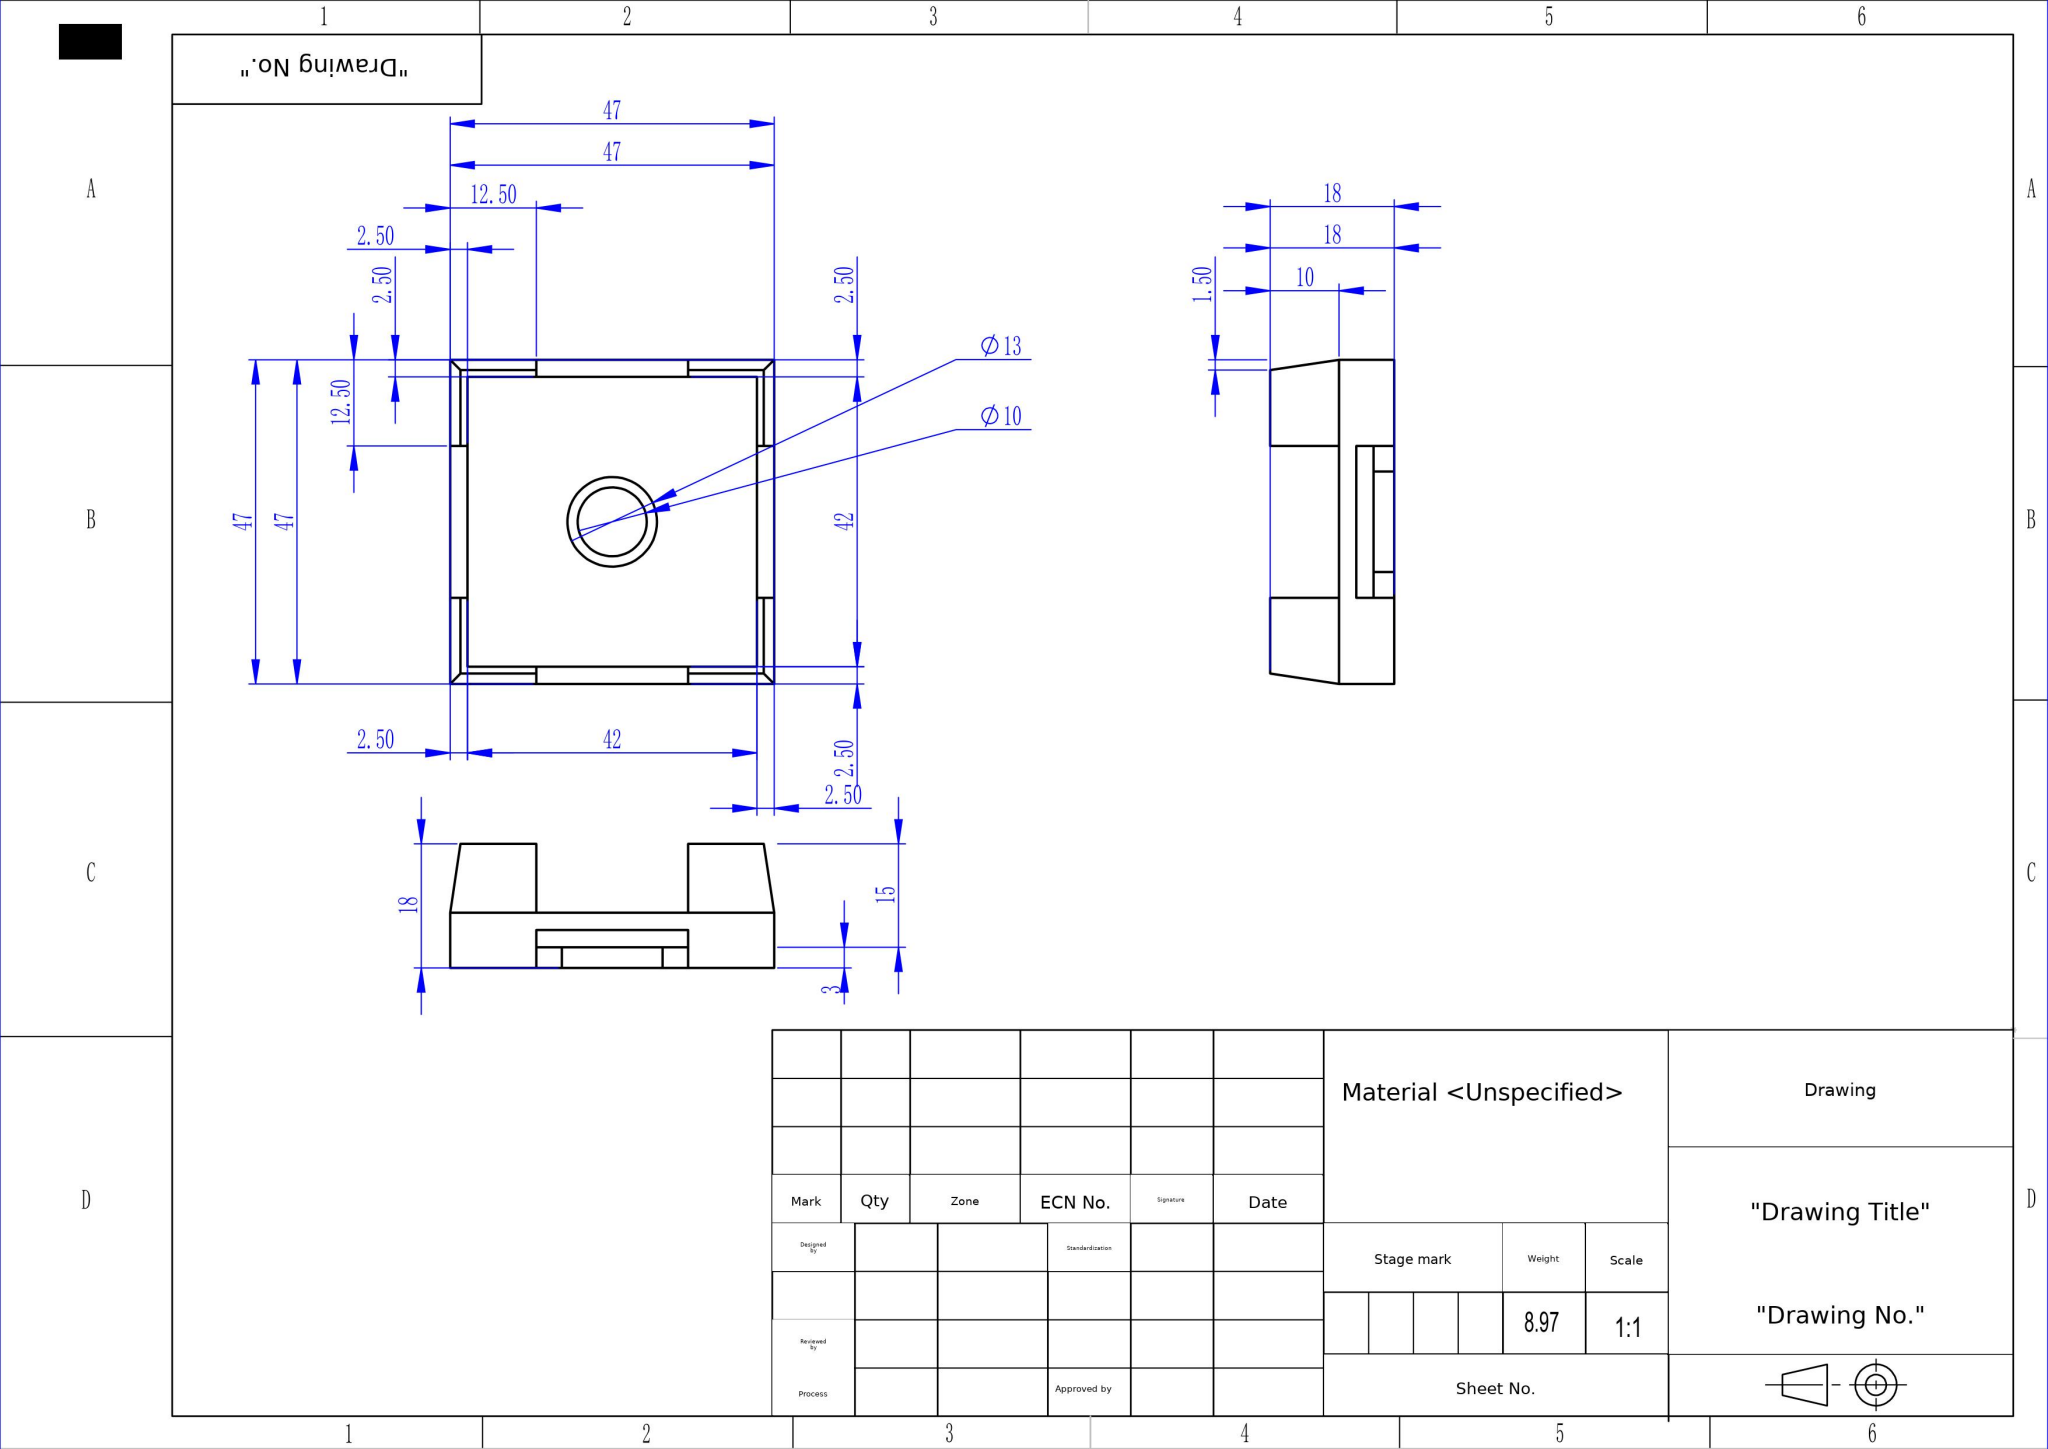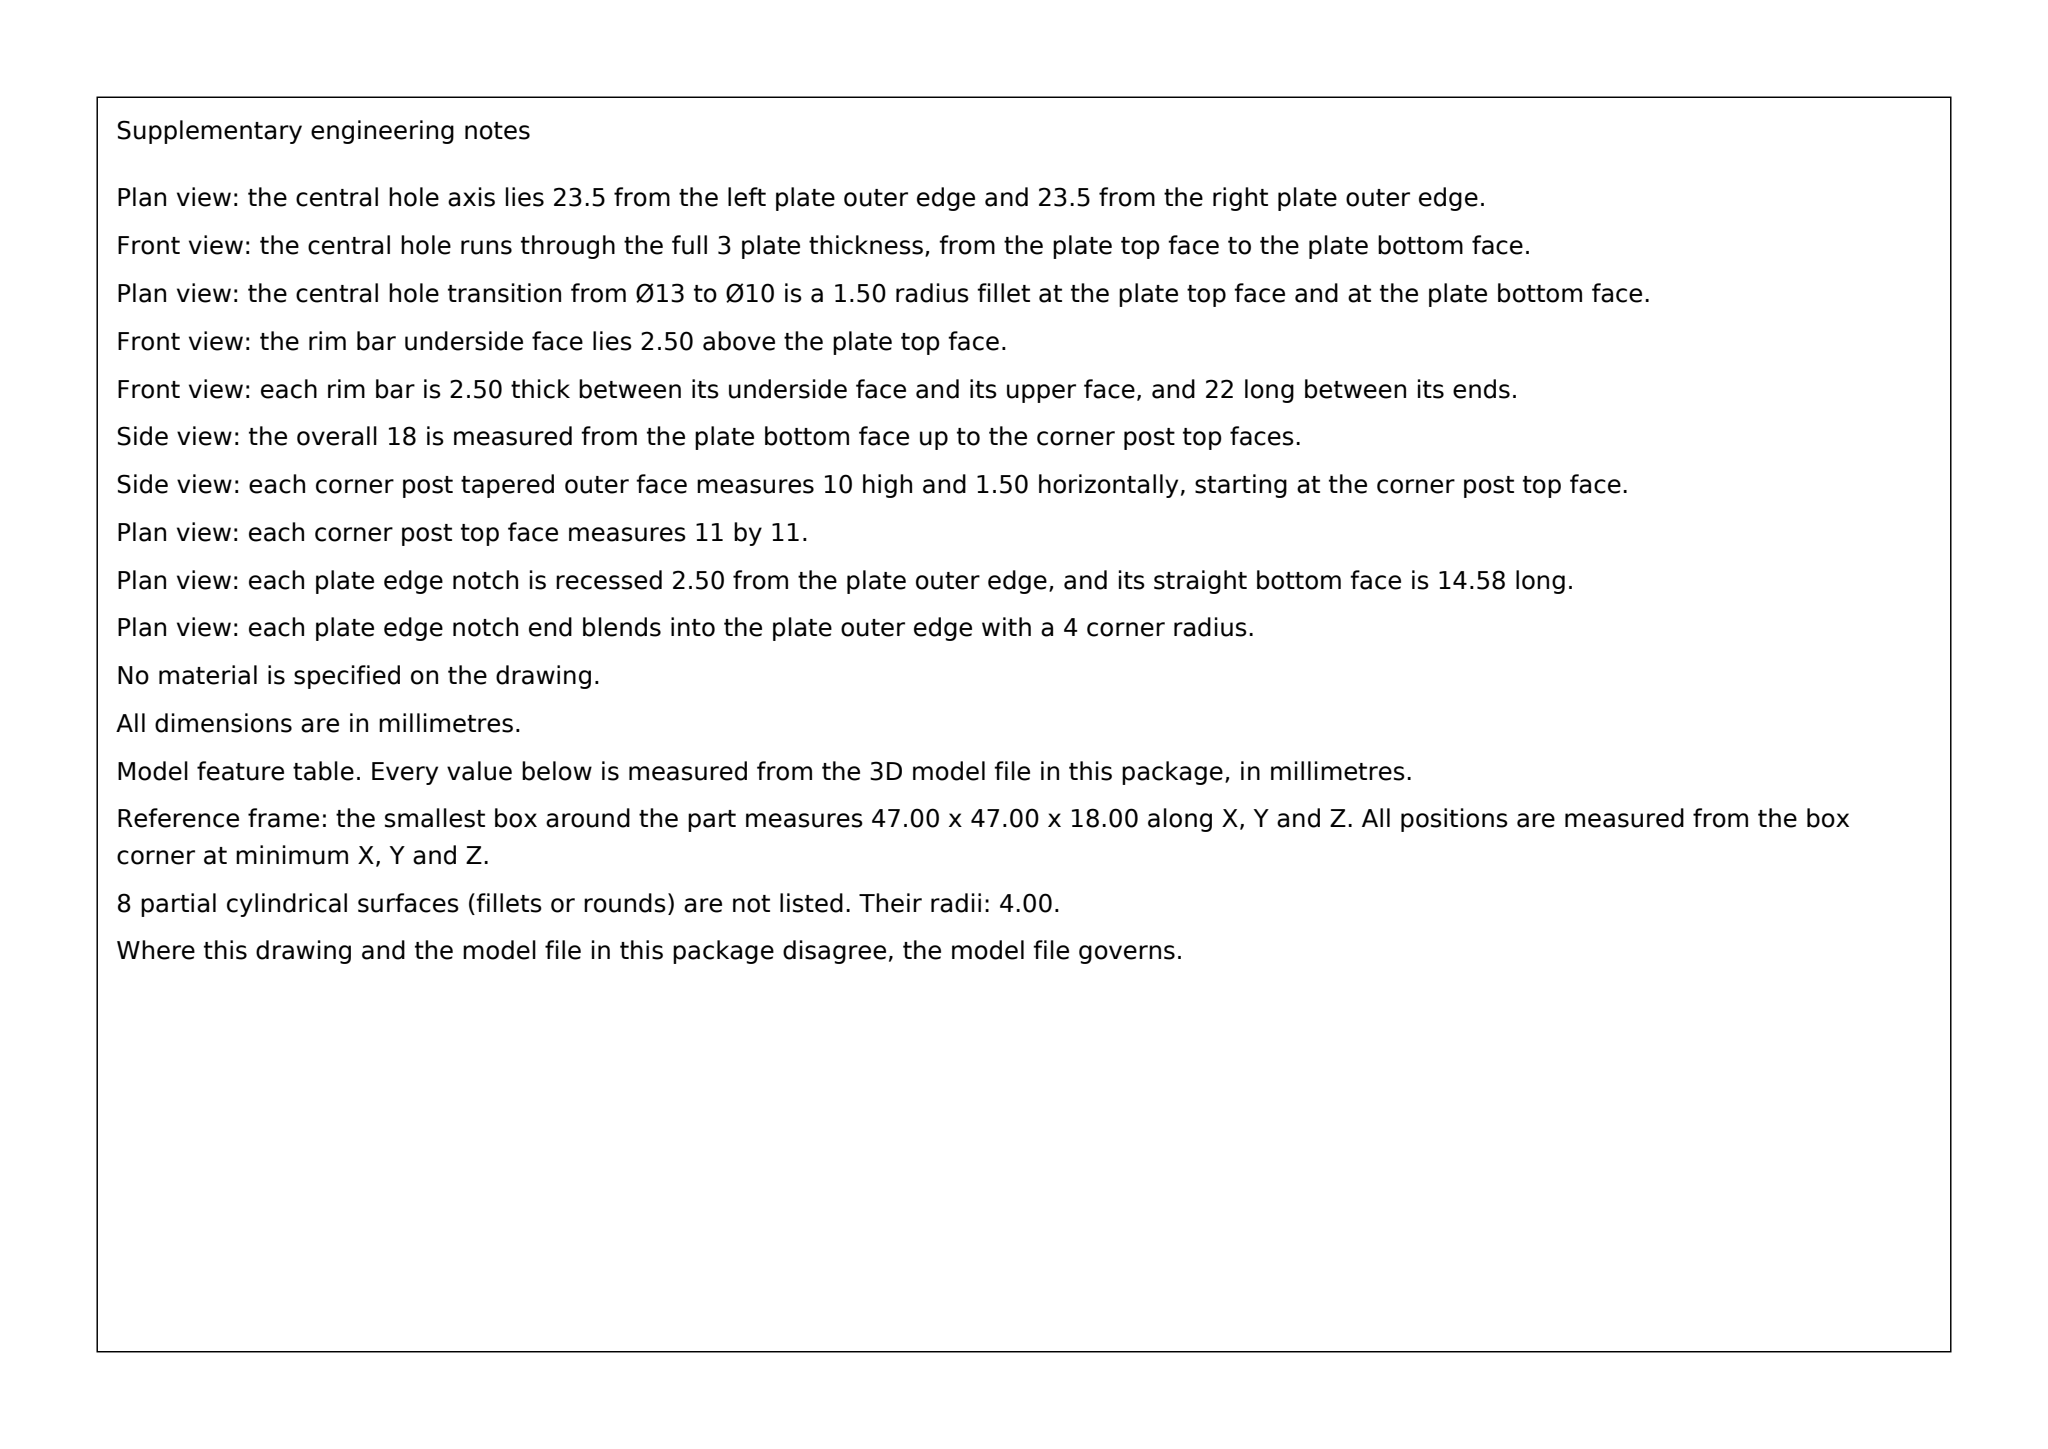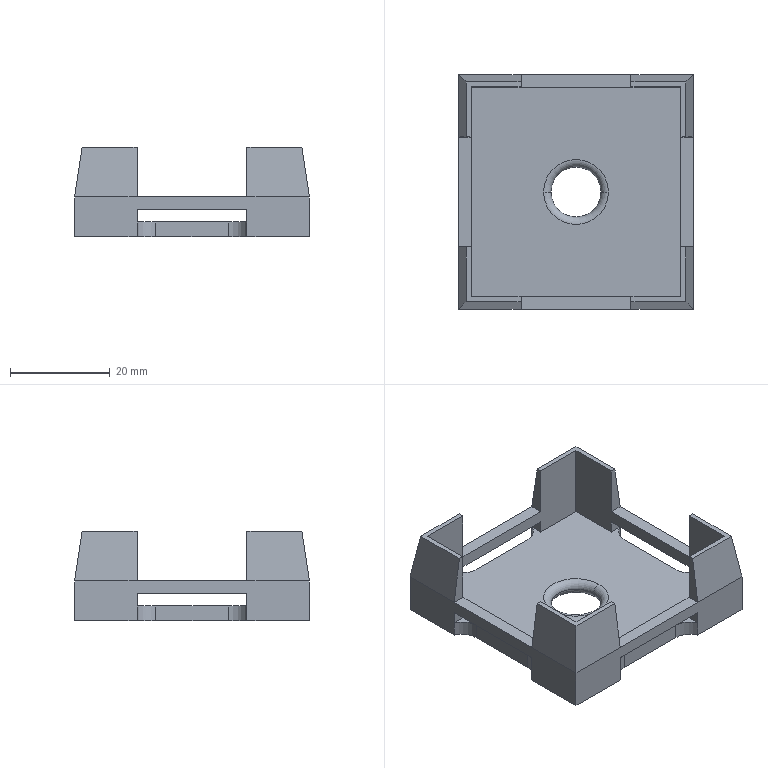Part | SolidWorks | mm | 1 solid | 62 faces | box 47 x 47 x 18 mm | volume 8965 mm3 | plane 50 | cylinder 8 | torus 4 | commonest cylinder face diameters 8 x8
Drawing notes:
4X CORNER PAD 12.50 SQ TOP Z18; SIDE RAILS 2.50 WD TOP Z8 | from the solid: X/Y planes 12.5 & 34.5 (4 faces ea) and 2.5/44.5; Z=18 (4 faces), Z=8 (4 faces), Z0 = bottom
RAIL INNER LEDGES AT Z5.50 FROM BOTTOM FACE | from the solid: Z plane at 5.5 with 4 coplanar faces between Z3 and Z8 levels
8X R4 SIDE SCALLOP 2.50 DP, DP 3 FROM BOTTOM, CL 16.21 & 30.79 | from the solid: 8X Ø8 Z-axis cylinders, length 3 from Z0, centres at -1.5/48.5 at 16.21 & 30.79
Ø10/Ø13 BORE CENTRED: 23.50 FROM EACH EDGE OF 47 X 47 | from the solid: bbox 47x47; bore axis on symmetry planes x=23.5, y=23.5 (fillet R1.5 x4 about centre)
Ø10 THRU 2.50 THK FLOOR; R1.50 BLEND AT TOP FACE = Ø13 | from the solid: z planes 3.0 and 5.5 give 2.5 floor thk; fillet_radii 1.5 -> 10+2(1.5)=13